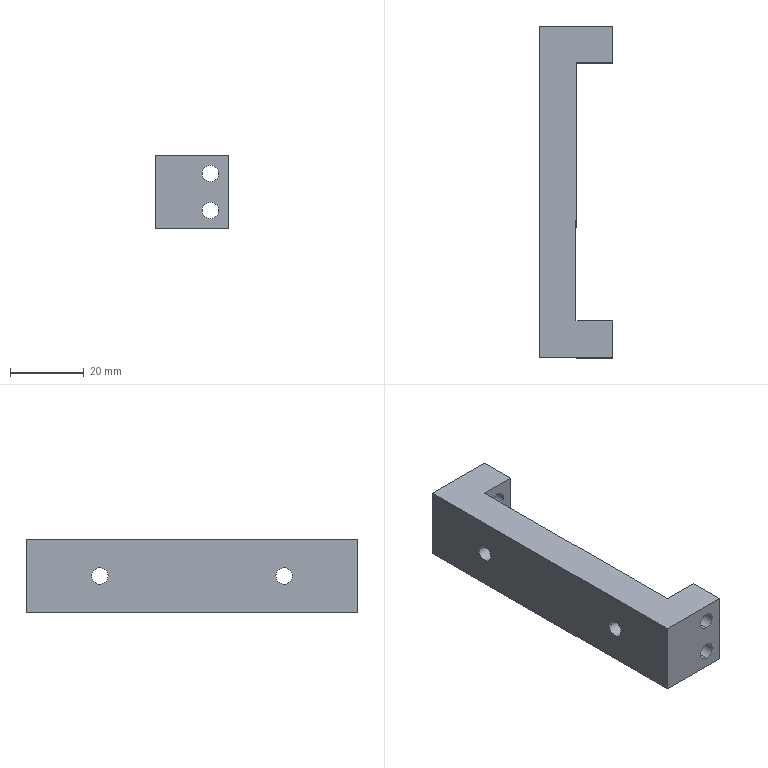Component | SolidWorks | U-shapedEpoxyBoard-2 | 1 solid | 28 faces | box 20 x 90 x 20 mm | volume 20743 mm3 | cylinder 16 | plane 12 | commonest cylinder face diameters 4.5 x12 8 x4
build123d program:
from build123d import *

# Parameters (mm, degrees)
SKETCH1_W                                       = 20
SKETCH1_H                                       = 20
BOSS_EXTRUDE1_DEPTH                             = 45
SKETCH2_W                                       = 70
SKETCH2_H                                       = 10
CUT_EXTRUDE1_DEPTH                              = 90
M4_HEX_SOCKET_HEAD_CAP_SCREW_CBORE1_D           = 4.5
M4_HEX_SOCKET_HEAD_CAP_SCREW_CBORE1_DEPTH       = 12.1
M4_HEX_SOCKET_HEAD_CAP_SCREW_CBORE1_CBORE_D     = 8
M4_HEX_SOCKET_HEAD_CAP_SCREW_CBORE1_CBORE_DEPTH = 4.4
M4_HEX_SOCKET_HEAD_CAP_SCREW_CBORE1_TIP         = 1.352
SKETCH4_R                                       = 2.25
CUT_EXTRUDE2_DEPTH                              = 90


with BuildPart() as part:
    # Sketch1 → Boss-Extrude1 (new, symmetric)
    with BuildSketch(Plane.XY):
        Rectangle(SKETCH1_W, SKETCH1_H)
    extrude(amount=BOSS_EXTRUDE1_DEPTH, both=True)

    # Sketch2 → Cut-Extrude1 (cut)
    with BuildSketch(Plane(origin=(10, 0, 0), x_dir=(0, 0, -1), z_dir=(1, 0, 0))):
        with Locations((0, -5)):
            Rectangle(SKETCH2_W, SKETCH2_H)
    extrude(amount=-CUT_EXTRUDE1_DEPTH, mode=Mode.SUBTRACT)

    # M4 Hex Socket Head Cap Screw CBORE1
    with Locations(Plane(origin=(0, 0, 25), x_dir=(0, 0, -1), z_dir=(0, -1, 0))):
        with Locations((0, 0), (50, 0)):
            CounterBoreHole(M4_HEX_SOCKET_HEAD_CAP_SCREW_CBORE1_D / 2, M4_HEX_SOCKET_HEAD_CAP_SCREW_CBORE1_CBORE_D / 2, M4_HEX_SOCKET_HEAD_CAP_SCREW_CBORE1_CBORE_DEPTH, depth=M4_HEX_SOCKET_HEAD_CAP_SCREW_CBORE1_DEPTH)
            with Locations((0, 0, -(M4_HEX_SOCKET_HEAD_CAP_SCREW_CBORE1_DEPTH + M4_HEX_SOCKET_HEAD_CAP_SCREW_CBORE1_TIP / 2))):  # 118° drill point
                Cone(0, M4_HEX_SOCKET_HEAD_CAP_SCREW_CBORE1_D / 2, M4_HEX_SOCKET_HEAD_CAP_SCREW_CBORE1_TIP, mode=Mode.SUBTRACT)

    # Sketch4 → Cut-Extrude2 (cut)
    with BuildSketch(Plane(origin=(0, 0, -45), x_dir=(-1, 0, 0), z_dir=(0, 0, -1))):
        with Locations((-5, -5)):
            Circle(SKETCH4_R)
        with Locations((5, -5)):
            Circle(SKETCH4_R)
    extrude(amount=-CUT_EXTRUDE2_DEPTH, mode=Mode.SUBTRACT)


solid = part.part

# Placed as in the assembly
solid = solid.moved(Location((-33.341, 37.185, -41.775), (90, 0, 90)))
STEP:
#1=COLOUR_RGB('',0.7922,0.8196,0.9333);
#2=FILL_AREA_STYLE_COLOUR('',#1);
#3=FILL_AREA_STYLE('',(#2));
#4=SURFACE_STYLE_FILL_AREA(#3);
#5=SURFACE_SIDE_STYLE('',(#4));
#6=SURFACE_STYLE_USAGE(.BOTH.,#5);
#7=PRESENTATION_STYLE_ASSIGNMENT((#6));
#8=CARTESIAN_POINT('',(-1.116,-0.3077,-1.753));
#9=VERTEX_POINT('',#8);
#10=CARTESIAN_POINT('',(-1.116,-0.3077,-1.93));
#11=VERTEX_POINT('',#10);
#12=CARTESIAN_POINT('',(-1.116,-0.3077,-1.842));
#13=DIRECTION('',(0.,1.,-0.));
#14=DIRECTION('',(0.,0.,-1.));
#15=AXIS2_PLACEMENT_3D('',#12,#13,#14);
#16=CIRCLE('',#15,0.08858);
#17=EDGE_CURVE('',#9,#11,#16,.T.);
#18=ORIENTED_EDGE('',*,*,#17,.F.);
#19=CARTESIAN_POINT('',(-1.116,0.08603,-1.753));
#20=VERTEX_POINT('',#19);
#21=CARTESIAN_POINT('',(-1.116,-0.3077,-1.753));
#22=DIRECTION('',(0.,1.,-0.));
#23=VECTOR('',#22,39.37);
#24=LINE('',#21,#23);
#25=EDGE_CURVE('',#9,#20,#24,.T.);
#26=ORIENTED_EDGE('',*,*,#25,.T.);
#27=CARTESIAN_POINT('',(-1.116,0.08603,-1.93));
#28=VERTEX_POINT('',#27);
#29=CARTESIAN_POINT('',(-1.116,0.08603,-1.842));
#30=DIRECTION('',(-0.,-1.,0.));
#31=DIRECTION('',(0.,0.,1.));
#32=AXIS2_PLACEMENT_3D('',#29,#30,#31);
#33=CIRCLE('',#32,0.08858);
#34=EDGE_CURVE('',#28,#20,#33,.T.);
#35=ORIENTED_EDGE('',*,*,#34,.F.);
#36=CARTESIAN_POINT('',(-1.116,-0.3077,-1.93));
#37=DIRECTION('',(0.,1.,-0.));
#38=VECTOR('',#37,39.37);
#39=LINE('',#36,#38);
#40=EDGE_CURVE('',#11,#28,#39,.T.);
#41=ORIENTED_EDGE('',*,*,#40,.F.);
#42=EDGE_LOOP('',(#18,#26,#35,#41));
#43=FACE_OUTER_BOUND('',#42,.T.);
#44=CARTESIAN_POINT('',(-1.116,-0.3077,-1.842));
#45=DIRECTION('',(0.,1.,-0.));
#46=DIRECTION('',(0.,0.,-1.));
#47=AXIS2_PLACEMENT_3D('',#44,#45,#46);
#48=CYLINDRICAL_SURFACE('',#47,0.08858);
#49=ADVANCED_FACE('',(#43),#48,.F.);
#50=CARTESIAN_POINT('',(-1.116,2.842,-1.753));
#51=VERTEX_POINT('',#50);
#52=CARTESIAN_POINT('',(-1.116,2.842,-1.93));
#53=VERTEX_POINT('',#52);
#54=CARTESIAN_POINT('',(-1.116,2.842,-1.842));
#55=DIRECTION('',(0.,1.,-0.));
#56=DIRECTION('',(0.,0.,-1.));
#57=AXIS2_PLACEMENT_3D('',#54,#55,#56);
#58=CIRCLE('',#57,0.08858);
#59=EDGE_CURVE('',#51,#53,#58,.T.);
#60=ORIENTED_EDGE('',*,*,#59,.F.);
#61=CARTESIAN_POINT('',(-1.116,3.236,-1.753));
#62=VERTEX_POINT('',#61);
#63=CARTESIAN_POINT('',(-1.116,-0.3077,-1.753));
#64=DIRECTION('',(0.,1.,-0.));
#65=VECTOR('',#64,39.37);
#66=LINE('',#63,#65);
#67=EDGE_CURVE('',#51,#62,#66,.T.);
#68=ORIENTED_EDGE('',*,*,#67,.T.);
#69=CARTESIAN_POINT('',(-1.116,3.236,-1.93));
#70=VERTEX_POINT('',#69);
#71=CARTESIAN_POINT('',(-1.116,3.236,-1.842));
#72=DIRECTION('',(0.,1.,-0.));
#73=DIRECTION('',(0.,0.,-1.));
#74=AXIS2_PLACEMENT_3D('',#71,#72,#73);
#75=CIRCLE('',#74,0.08858);
#76=EDGE_CURVE('',#62,#70,#75,.T.);
#77=ORIENTED_EDGE('',*,*,#76,.T.);
#78=CARTESIAN_POINT('',(-1.116,-0.3077,-1.93));
#79=DIRECTION('',(0.,1.,-0.));
#80=VECTOR('',#79,39.37);
#81=LINE('',#78,#80);
#82=EDGE_CURVE('',#53,#70,#81,.T.);
#83=ORIENTED_EDGE('',*,*,#82,.F.);
#84=EDGE_LOOP('',(#60,#68,#77,#83));
#85=FACE_OUTER_BOUND('',#84,.T.);
#86=CARTESIAN_POINT('',(-1.116,-0.3077,-1.842));
#87=DIRECTION('',(0.,1.,-0.));
#88=DIRECTION('',(0.,0.,-1.));
#89=AXIS2_PLACEMENT_3D('',#86,#87,#88);
#90=CYLINDRICAL_SURFACE('',#89,0.08858);
#91=ADVANCED_FACE('',(#85),#90,.F.);
#92=CARTESIAN_POINT('',(-1.116,-0.3077,-1.359));
#93=VERTEX_POINT('',#92);
#94=CARTESIAN_POINT('',(-1.116,-0.3077,-1.536));
#95=VERTEX_POINT('',#94);
#96=CARTESIAN_POINT('',(-1.116,-0.3077,-1.448));
#97=DIRECTION('',(0.,1.,-0.));
#98=DIRECTION('',(0.,0.,-1.));
#99=AXIS2_PLACEMENT_3D('',#96,#97,#98);
#100=CIRCLE('',#99,0.08858);
#101=EDGE_CURVE('',#93,#95,#100,.T.);
#102=ORIENTED_EDGE('',*,*,#101,.F.);
#103=CARTESIAN_POINT('',(-1.116,0.08603,-1.359));
#104=VERTEX_POINT('',#103);
#105=CARTESIAN_POINT('',(-1.116,-0.3077,-1.359));
#106=DIRECTION('',(0.,1.,-0.));
#107=VECTOR('',#106,39.37);
#108=LINE('',#105,#107);
#109=EDGE_CURVE('',#93,#104,#108,.T.);
#110=ORIENTED_EDGE('',*,*,#109,.T.);
#111=CARTESIAN_POINT('',(-1.116,0.08603,-1.536));
#112=VERTEX_POINT('',#111);
#113=CARTESIAN_POINT('',(-1.116,0.08603,-1.448));
#114=DIRECTION('',(-0.,-1.,0.));
#115=DIRECTION('',(0.,0.,1.));
#116=AXIS2_PLACEMENT_3D('',#113,#114,#115);
#117=CIRCLE('',#116,0.08858);
#118=EDGE_CURVE('',#112,#104,#117,.T.);
#119=ORIENTED_EDGE('',*,*,#118,.F.);
#120=CARTESIAN_POINT('',(-1.116,-0.3077,-1.536));
#121=DIRECTION('',(0.,1.,-0.));
#122=VECTOR('',#121,39.37);
#123=LINE('',#120,#122);
#124=EDGE_CURVE('',#95,#112,#123,.T.);
#125=ORIENTED_EDGE('',*,*,#124,.F.);
#126=EDGE_LOOP('',(#102,#110,#119,#125));
#127=FACE_OUTER_BOUND('',#126,.T.);
#128=CARTESIAN_POINT('',(-1.116,-0.3077,-1.448));
#129=DIRECTION('',(0.,1.,-0.));
#130=DIRECTION('',(0.,0.,-1.));
#131=AXIS2_PLACEMENT_3D('',#128,#129,#130);
#132=CYLINDRICAL_SURFACE('',#131,0.08858);
#133=ADVANCED_FACE('',(#127),#132,.F.);
#134=CARTESIAN_POINT('',(-1.116,2.842,-1.359));
#135=VERTEX_POINT('',#134);
#136=CARTESIAN_POINT('',(-1.116,2.842,-1.536));
#137=VERTEX_POINT('',#136);
#138=CARTESIAN_POINT('',(-1.116,2.842,-1.448));
#139=DIRECTION('',(0.,1.,-0.));
#140=DIRECTION('',(0.,0.,-1.));
#141=AXIS2_PLACEMENT_3D('',#138,#139,#140);
#142=CIRCLE('',#141,0.08858);
#143=EDGE_CURVE('',#135,#137,#142,.T.);
#144=ORIENTED_EDGE('',*,*,#143,.F.);
#145=CARTESIAN_POINT('',(-1.116,3.236,-1.359));
#146=VERTEX_POINT('',#145);
#147=CARTESIAN_POINT('',(-1.116,-0.3077,-1.359));
#148=DIRECTION('',(0.,1.,-0.));
#149=VECTOR('',#148,39.37);
#150=LINE('',#147,#149);
#151=EDGE_CURVE('',#135,#146,#150,.T.);
#152=ORIENTED_EDGE('',*,*,#151,.T.);
#153=CARTESIAN_POINT('',(-1.116,3.236,-1.536));
#154=VERTEX_POINT('',#153);
#155=CARTESIAN_POINT('',(-1.116,3.236,-1.448));
#156=DIRECTION('',(0.,1.,-0.));
#157=DIRECTION('',(0.,0.,-1.));
#158=AXIS2_PLACEMENT_3D('',#155,#156,#157);
#159=CIRCLE('',#158,0.08858);
#160=EDGE_CURVE('',#146,#154,#159,.T.);
#161=ORIENTED_EDGE('',*,*,#160,.T.);
#162=CARTESIAN_POINT('',(-1.116,-0.3077,-1.536));
#163=DIRECTION('',(0.,1.,-0.));
#164=VECTOR('',#163,39.37);
#165=LINE('',#162,#164);
#166=EDGE_CURVE('',#137,#154,#165,.T.);
#167=ORIENTED_EDGE('',*,*,#166,.F.);
#168=EDGE_LOOP('',(#144,#152,#161,#167));
#169=FACE_OUTER_BOUND('',#168,.T.);
#170=CARTESIAN_POINT('',(-1.116,-0.3077,-1.448));
#171=DIRECTION('',(0.,1.,-0.));
#172=DIRECTION('',(0.,0.,-1.));
#173=AXIS2_PLACEMENT_3D('',#170,#171,#172);
#174=CYLINDRICAL_SURFACE('',#173,0.08858);
#175=ADVANCED_FACE('',(#169),#174,.F.);
#176=CARTESIAN_POINT('',(-1.486,0.3223,-1.645));
#177=VERTEX_POINT('',#176);
#178=CARTESIAN_POINT('',(-1.486,0.6372,-1.645));
#179=VERTEX_POINT('',#178);
#180=CARTESIAN_POINT('',(-1.486,0.4797,-1.645));
#181=DIRECTION('',(1.,-0.,-0.));
#182=DIRECTION('',(0.,1.,0.));
#183=AXIS2_PLACEMENT_3D('',#180,#181,#182);
#184=CIRCLE('',#183,0.1575);
#185=EDGE_CURVE('',#177,#179,#184,.T.);
#186=ORIENTED_EDGE('',*,*,#185,.F.);
#187=CARTESIAN_POINT('',(-1.313,0.3223,-1.645));
#188=VERTEX_POINT('',#187);
#189=CARTESIAN_POINT('',(-1.313,0.3223,-1.645));
#190=DIRECTION('',(1.,-0.,-0.));
#191=VECTOR('',#190,39.37);
#192=LINE('',#189,#191);
#193=EDGE_CURVE('',#177,#188,#192,.T.);
#194=ORIENTED_EDGE('',*,*,#193,.T.);
#195=CARTESIAN_POINT('',(-1.313,0.6372,-1.645));
#196=VERTEX_POINT('',#195);
#197=CARTESIAN_POINT('',(-1.313,0.4797,-1.645));
#198=DIRECTION('',(1.,-0.,-0.));
#199=DIRECTION('',(0.,1.,0.));
#200=AXIS2_PLACEMENT_3D('',#197,#198,#199);
#201=CIRCLE('',#200,0.1575);
#202=EDGE_CURVE('',#188,#196,#201,.T.);
#203=ORIENTED_EDGE('',*,*,#202,.T.);
#204=CARTESIAN_POINT('',(-1.313,0.6372,-1.645));
#205=DIRECTION('',(1.,-0.,-0.));
#206=VECTOR('',#205,39.37);
#207=LINE('',#204,#206);
#208=EDGE_CURVE('',#179,#196,#207,.T.);
#209=ORIENTED_EDGE('',*,*,#208,.F.);
#210=EDGE_LOOP('',(#186,#194,#203,#209));
#211=FACE_OUTER_BOUND('',#210,.T.);
#212=CARTESIAN_POINT('',(-1.313,0.4797,-1.645));
#213=DIRECTION('',(1.,-0.,-0.));
#214=DIRECTION('',(0.,1.,0.));
#215=AXIS2_PLACEMENT_3D('',#212,#213,#214);
#216=CYLINDRICAL_SURFACE('',#215,0.1575);
#217=ADVANCED_FACE('',(#211),#216,.F.);
#218=CARTESIAN_POINT('',(-1.706,0.3912,-1.645));
#219=VERTEX_POINT('',#218);
#220=CARTESIAN_POINT('',(-1.706,0.5683,-1.645));
#221=VERTEX_POINT('',#220);
#222=CARTESIAN_POINT('',(-1.706,0.4797,-1.645));
#223=DIRECTION('',(1.,-0.,-0.));
#224=DIRECTION('',(0.,1.,0.));
#225=AXIS2_PLACEMENT_3D('',#222,#223,#224);
#226=CIRCLE('',#225,0.08858);
#227=EDGE_CURVE('',#219,#221,#226,.T.);
#228=ORIENTED_EDGE('',*,*,#227,.F.);
#229=CARTESIAN_POINT('',(-1.486,0.3912,-1.645));
#230=VERTEX_POINT('',#229);
#231=CARTESIAN_POINT('',(-1.313,0.3912,-1.645));
#232=DIRECTION('',(1.,-0.,-0.));
#233=VECTOR('',#232,39.37);
#234=LINE('',#231,#233);
#235=EDGE_CURVE('',#219,#230,#234,.T.);
#236=ORIENTED_EDGE('',*,*,#235,.T.);
#237=CARTESIAN_POINT('',(-1.486,0.5683,-1.645));
#238=VERTEX_POINT('',#237);
#239=CARTESIAN_POINT('',(-1.486,0.4797,-1.645));
#240=DIRECTION('',(1.,-0.,-0.));
#241=DIRECTION('',(0.,1.,0.));
#242=AXIS2_PLACEMENT_3D('',#239,#240,#241);
#243=CIRCLE('',#242,0.08858);
#244=EDGE_CURVE('',#230,#238,#243,.T.);
#245=ORIENTED_EDGE('',*,*,#244,.T.);
#246=CARTESIAN_POINT('',(-1.313,0.5683,-1.645));
#247=DIRECTION('',(1.,-0.,-0.));
#248=VECTOR('',#247,39.37);
#249=LINE('',#246,#248);
#250=EDGE_CURVE('',#221,#238,#249,.T.);
#251=ORIENTED_EDGE('',*,*,#250,.F.);
#252=EDGE_LOOP('',(#228,#236,#245,#251));
#253=FACE_OUTER_BOUND('',#252,.T.);
#254=CARTESIAN_POINT('',(-1.313,0.4797,-1.645));
#255=DIRECTION('',(1.,-0.,-0.));
#256=DIRECTION('',(0.,1.,0.));
#257=AXIS2_PLACEMENT_3D('',#254,#255,#256);
#258=CYLINDRICAL_SURFACE('',#257,0.08858);
#259=ADVANCED_FACE('',(#253),#258,.F.);
#260=CARTESIAN_POINT('',(-1.486,2.291,-1.645));
#261=VERTEX_POINT('',#260);
#262=CARTESIAN_POINT('',(-1.486,2.606,-1.645));
#263=VERTEX_POINT('',#262);
#264=CARTESIAN_POINT('',(-1.486,2.448,-1.645));
#265=DIRECTION('',(1.,-0.,-0.));
#266=DIRECTION('',(0.,1.,0.));
#267=AXIS2_PLACEMENT_3D('',#264,#265,#266);
#268=CIRCLE('',#267,0.1575);
#269=EDGE_CURVE('',#261,#263,#268,.T.);
#270=ORIENTED_EDGE('',*,*,#269,.F.);
#271=CARTESIAN_POINT('',(-1.313,2.291,-1.645));
#272=VERTEX_POINT('',#271);
#273=CARTESIAN_POINT('',(-1.313,2.291,-1.645));
#274=DIRECTION('',(1.,-0.,-0.));
#275=VECTOR('',#274,39.37);
#276=LINE('',#273,#275);
#277=EDGE_CURVE('',#261,#272,#276,.T.);
#278=ORIENTED_EDGE('',*,*,#277,.T.);
#279=CARTESIAN_POINT('',(-1.313,2.606,-1.645));
#280=VERTEX_POINT('',#279);
#281=CARTESIAN_POINT('',(-1.313,2.448,-1.645));
#282=DIRECTION('',(1.,-0.,-0.));
#283=DIRECTION('',(0.,1.,0.));
#284=AXIS2_PLACEMENT_3D('',#281,#282,#283);
#285=CIRCLE('',#284,0.1575);
#286=EDGE_CURVE('',#272,#280,#285,.T.);
#287=ORIENTED_EDGE('',*,*,#286,.T.);
#288=CARTESIAN_POINT('',(-1.313,2.606,-1.645));
#289=DIRECTION('',(1.,-0.,-0.));
#290=VECTOR('',#289,39.37);
#291=LINE('',#288,#290);
#292=EDGE_CURVE('',#263,#280,#291,.T.);
#293=ORIENTED_EDGE('',*,*,#292,.F.);
#294=EDGE_LOOP('',(#270,#278,#287,#293));
#295=FACE_OUTER_BOUND('',#294,.T.);
#296=CARTESIAN_POINT('',(-1.313,2.448,-1.645));
#297=DIRECTION('',(1.,-0.,-0.));
#298=DIRECTION('',(0.,1.,0.));
#299=AXIS2_PLACEMENT_3D('',#296,#297,#298);
#300=CYLINDRICAL_SURFACE('',#299,0.1575);
#301=ADVANCED_FACE('',(#295),#300,.F.);
#302=CARTESIAN_POINT('',(-1.706,2.36,-1.645));
#303=VERTEX_POINT('',#302);
#304=CARTESIAN_POINT('',(-1.706,2.537,-1.645));
#305=VERTEX_POINT('',#304);
#306=CARTESIAN_POINT('',(-1.706,2.448,-1.645));
#307=DIRECTION('',(1.,-0.,-0.));
#308=DIRECTION('',(0.,1.,0.));
#309=AXIS2_PLACEMENT_3D('',#306,#307,#308);
#310=CIRCLE('',#309,0.08858);
#311=EDGE_CURVE('',#303,#305,#310,.T.);
#312=ORIENTED_EDGE('',*,*,#311,.F.);
#313=CARTESIAN_POINT('',(-1.486,2.36,-1.645));
#314=VERTEX_POINT('',#313);
#315=CARTESIAN_POINT('',(-1.313,2.36,-1.645));
#316=DIRECTION('',(1.,-0.,-0.));
#317=VECTOR('',#316,39.37);
#318=LINE('',#315,#317);
#319=EDGE_CURVE('',#303,#314,#318,.T.);
#320=ORIENTED_EDGE('',*,*,#319,.T.);
#321=CARTESIAN_POINT('',(-1.486,2.537,-1.645));
#322=VERTEX_POINT('',#321);
#323=CARTESIAN_POINT('',(-1.486,2.448,-1.645));
#324=DIRECTION('',(1.,-0.,-0.));
#325=DIRECTION('',(0.,1.,0.));
#326=AXIS2_PLACEMENT_3D('',#323,#324,#325);
#327=CIRCLE('',#326,0.08858);
#328=EDGE_CURVE('',#314,#322,#327,.T.);
#329=ORIENTED_EDGE('',*,*,#328,.T.);
#330=CARTESIAN_POINT('',(-1.313,2.537,-1.645));
#331=DIRECTION('',(1.,-0.,-0.));
#332=VECTOR('',#331,39.37);
#333=LINE('',#330,#332);
#334=EDGE_CURVE('',#305,#322,#333,.T.);
#335=ORIENTED_EDGE('',*,*,#334,.F.);
#336=EDGE_LOOP('',(#312,#320,#329,#335));
#337=FACE_OUTER_BOUND('',#336,.T.);
#338=CARTESIAN_POINT('',(-1.313,2.448,-1.645));
#339=DIRECTION('',(1.,-0.,-0.));
#340=DIRECTION('',(0.,1.,0.));
#341=AXIS2_PLACEMENT_3D('',#338,#339,#340);
#342=CYLINDRICAL_SURFACE('',#341,0.08858);
#343=ADVANCED_FACE('',(#337),#342,.F.);
#344=CARTESIAN_POINT('',(-0.919,-0.3077,-2.038));
#345=VERTEX_POINT('',#344);
#346=CARTESIAN_POINT('',(-0.919,0.08603,-2.038));
#347=VERTEX_POINT('',#346);
#348=CARTESIAN_POINT('',(-0.919,-0.3077,-2.038));
#349=DIRECTION('',(0.,1.,-0.));
#350=VECTOR('',#349,39.37);
#351=LINE('',#348,#350);
#352=EDGE_CURVE('',#345,#347,#351,.T.);
#353=ORIENTED_EDGE('',*,*,#352,.T.);
#354=CARTESIAN_POINT('',(-0.919,0.08603,-1.251));
#355=VERTEX_POINT('',#354);
#356=CARTESIAN_POINT('',(-0.919,0.08603,-4.794));
#357=DIRECTION('',(0.,0.,1.));
#358=VECTOR('',#357,39.37);
#359=LINE('',#356,#358);
#360=EDGE_CURVE('',#347,#355,#359,.T.);
#361=ORIENTED_EDGE('',*,*,#360,.T.);
#362=CARTESIAN_POINT('',(-0.919,-0.3077,-1.251));
#363=VERTEX_POINT('',#362);
#364=CARTESIAN_POINT('',(-0.919,-0.3077,-1.251));
#365=DIRECTION('',(0.,1.,-0.));
#366=VECTOR('',#365,39.37);
#367=LINE('',#364,#366);
#368=EDGE_CURVE('',#363,#355,#367,.T.);
#369=ORIENTED_EDGE('',*,*,#368,.F.);
#370=CARTESIAN_POINT('',(-0.919,-0.3077,-2.038));
#371=DIRECTION('',(0.,0.,1.));
#372=VECTOR('',#371,39.37);
#373=LINE('',#370,#372);
#374=EDGE_CURVE('',#345,#363,#373,.T.);
#375=ORIENTED_EDGE('',*,*,#374,.F.);
#376=EDGE_LOOP('',(#353,#361,#369,#375));
#377=FACE_OUTER_BOUND('',#376,.T.);
#378=CARTESIAN_POINT('',(-0.919,-0.3077,-2.038));
#379=DIRECTION('',(-1.,0.,0.));
#380=DIRECTION('',(-0.,-1.,0.));
#381=AXIS2_PLACEMENT_3D('',#378,#379,#380);
#382=PLANE('',#381);
#383=ADVANCED_FACE('',(#377),#382,.F.);
#384=CARTESIAN_POINT('',(-1.313,2.842,-2.038));
#385=VERTEX_POINT('',#384);
#386=CARTESIAN_POINT('',(-1.313,0.08603,-2.038));
#387=VERTEX_POINT('',#386);
#388=CARTESIAN_POINT('',(-1.313,-0.3077,-2.038));
#389=DIRECTION('',(-0.,-1.,0.));
#390=VECTOR('',#389,39.37);
#391=LINE('',#388,#390);
#392=EDGE_CURVE('',#385,#387,#391,.T.);
#393=ORIENTED_EDGE('',*,*,#392,.T.);
#394=CARTESIAN_POINT('',(-1.706,0.08603,-2.038));
#395=DIRECTION('',(1.,-0.,-0.));
#396=VECTOR('',#395,39.37);
#397=LINE('',#394,#396);
#398=EDGE_CURVE('',#387,#347,#397,.T.);
#399=ORIENTED_EDGE('',*,*,#398,.T.);
#400=ORIENTED_EDGE('',*,*,#352,.F.);
#401=CARTESIAN_POINT('',(-1.706,-0.3077,-2.038));
#402=VERTEX_POINT('',#401);
#403=CARTESIAN_POINT('',(-1.706,-0.3077,-2.038));
#404=DIRECTION('',(1.,-0.,-0.));
#405=VECTOR('',#404,39.37);
#406=LINE('',#403,#405);
#407=EDGE_CURVE('',#402,#345,#406,.T.);
#408=ORIENTED_EDGE('',*,*,#407,.F.);
#409=CARTESIAN_POINT('',(-1.706,3.236,-2.038));
#410=VERTEX_POINT('',#409);
#411=CARTESIAN_POINT('',(-1.706,-0.3077,-2.038));
#412=DIRECTION('',(0.,1.,-0.));
#413=VECTOR('',#412,39.37);
#414=LINE('',#411,#413);
#415=EDGE_CURVE('',#402,#410,#414,.T.);
#416=ORIENTED_EDGE('',*,*,#415,.T.);
#417=CARTESIAN_POINT('',(-0.919,3.236,-2.038));
#418=VERTEX_POINT('',#417);
#419=CARTESIAN_POINT('',(-1.706,3.236,-2.038));
#420=DIRECTION('',(1.,-0.,-0.));
#421=VECTOR('',#420,39.37);
#422=LINE('',#419,#421);
#423=EDGE_CURVE('',#410,#418,#422,.T.);
#424=ORIENTED_EDGE('',*,*,#423,.T.);
#425=CARTESIAN_POINT('',(-0.919,2.842,-2.038));
#426=VERTEX_POINT('',#425);
#427=CARTESIAN_POINT('',(-0.919,-0.3077,-2.038));
#428=DIRECTION('',(0.,1.,-0.));
#429=VECTOR('',#428,39.37);
#430=LINE('',#427,#429);
#431=EDGE_CURVE('',#426,#418,#430,.T.);
#432=ORIENTED_EDGE('',*,*,#431,.F.);
#433=CARTESIAN_POINT('',(-1.706,2.842,-2.038));
#434=DIRECTION('',(-1.,0.,0.));
#435=VECTOR('',#434,39.37);
#436=LINE('',#433,#435);
#437=EDGE_CURVE('',#426,#385,#436,.T.);
#438=ORIENTED_EDGE('',*,*,#437,.T.);
#439=EDGE_LOOP('',(#393,#399,#400,#408,#416,#424,#432,#438));
#440=FACE_OUTER_BOUND('',#439,.T.);
#441=CARTESIAN_POINT('',(-1.706,-0.3077,-2.038));
#442=DIRECTION('',(0.,0.,1.));
#443=DIRECTION('',(-1.,0.,0.));
#444=AXIS2_PLACEMENT_3D('',#441,#442,#443);
#445=PLANE('',#444);
#446=ADVANCED_FACE('',(#440),#445,.F.);
#447=CARTESIAN_POINT('',(-0.919,2.842,-1.251));
#448=VERTEX_POINT('',#447);
#449=CARTESIAN_POINT('',(-0.919,3.236,-1.251));
#450=VERTEX_POINT('',#449);
#451=CARTESIAN_POINT('',(-0.919,-0.3077,-1.251));
#452=DIRECTION('',(0.,1.,-0.));
#453=VECTOR('',#452,39.37);
#454=LINE('',#451,#453);
#455=EDGE_CURVE('',#448,#450,#454,.T.);
#456=ORIENTED_EDGE('',*,*,#455,.F.);
#457=CARTESIAN_POINT('',(-0.919,2.842,-4.794));
#458=DIRECTION('',(0.,0.,1.));
#459=VECTOR('',#458,39.37);
#460=LINE('',#457,#459);
#461=EDGE_CURVE('',#426,#448,#460,.T.);
#462=ORIENTED_EDGE('',*,*,#461,.F.);
#463=ORIENTED_EDGE('',*,*,#431,.T.);
#464=CARTESIAN_POINT('',(-0.919,3.236,-2.038));
#465=DIRECTION('',(0.,0.,1.));
#466=VECTOR('',#465,39.37);
#467=LINE('',#464,#466);
#468=EDGE_CURVE('',#418,#450,#467,.T.);
#469=ORIENTED_EDGE('',*,*,#468,.T.);
#470=EDGE_LOOP('',(#456,#462,#463,#469));
#471=FACE_OUTER_BOUND('',#470,.T.);
#472=CARTESIAN_POINT('',(-0.919,-0.3077,-2.038));
#473=DIRECTION('',(-1.,0.,0.));
#474=DIRECTION('',(-0.,-1.,0.));
#475=AXIS2_PLACEMENT_3D('',#472,#473,#474);
#476=PLANE('',#475);
#477=ADVANCED_FACE('',(#471),#476,.F.);
#478=ORIENTED_EDGE('',*,*,#368,.T.);
#479=CARTESIAN_POINT('',(-1.313,0.08603,-1.251));
#480=VERTEX_POINT('',#479);
#481=CARTESIAN_POINT('',(-0.919,0.08603,-1.251));
#482=DIRECTION('',(1.,-0.,-0.));
#483=VECTOR('',#482,39.37);
#484=LINE('',#481,#483);
#485=EDGE_CURVE('',#480,#355,#484,.T.);
#486=ORIENTED_EDGE('',*,*,#485,.F.);
#487=CARTESIAN_POINT('',(-1.313,2.842,-1.251));
#488=VERTEX_POINT('',#487);
#489=CARTESIAN_POINT('',(-1.313,0.08603,-1.251));
#490=DIRECTION('',(-0.,-1.,0.));
#491=VECTOR('',#490,39.37);
#492=LINE('',#489,#491);
#493=EDGE_CURVE('',#488,#480,#492,.T.);
#494=ORIENTED_EDGE('',*,*,#493,.F.);
#495=CARTESIAN_POINT('',(-0.919,2.842,-1.251));
#496=DIRECTION('',(-1.,0.,0.));
#497=VECTOR('',#496,39.37);
#498=LINE('',#495,#497);
#499=EDGE_CURVE('',#448,#488,#498,.T.);
#500=ORIENTED_EDGE('',*,*,#499,.F.);
#501=ORIENTED_EDGE('',*,*,#455,.T.);
#502=CARTESIAN_POINT('',(-1.706,3.236,-1.251));
#503=VERTEX_POINT('',#502);
#504=CARTESIAN_POINT('',(-1.706,3.236,-1.251));
#505=DIRECTION('',(-1.,0.,0.));
#506=VECTOR('',#505,39.37);
#507=LINE('',#504,#506);
#508=EDGE_CURVE('',#450,#503,#507,.T.);
#509=ORIENTED_EDGE('',*,*,#508,.T.);
#510=CARTESIAN_POINT('',(-1.706,-0.3077,-1.251));
#511=VERTEX_POINT('',#510);
#512=CARTESIAN_POINT('',(-1.706,-0.3077,-1.251));
#513=DIRECTION('',(0.,1.,-0.));
#514=VECTOR('',#513,39.37);
#515=LINE('',#512,#514);
#516=EDGE_CURVE('',#511,#503,#515,.T.);
#517=ORIENTED_EDGE('',*,*,#516,.F.);
#518=CARTESIAN_POINT('',(-1.706,-0.3077,-1.251));
#519=DIRECTION('',(-1.,0.,0.));
#520=VECTOR('',#519,39.37);
#521=LINE('',#518,#520);
#522=EDGE_CURVE('',#363,#511,#521,.T.);
#523=ORIENTED_EDGE('',*,*,#522,.F.);
#524=EDGE_LOOP('',(#478,#486,#494,#500,#501,#509,#517,#523));
#525=FACE_OUTER_BOUND('',#524,.T.);
#526=CARTESIAN_POINT('',(-1.706,-0.3077,-1.251));
#527=DIRECTION('',(-0.,-0.,-1.));
#528=DIRECTION('',(-0.,-1.,0.));
#529=AXIS2_PLACEMENT_3D('',#526,#527,#528);
#530=PLANE('',#529);
#531=ADVANCED_FACE('',(#525),#530,.F.);
#532=CARTESIAN_POINT('',(-1.706,0.4797,-1.645));
#533=DIRECTION('',(1.,-0.,-0.));
#534=DIRECTION('',(0.,1.,0.));
#535=AXIS2_PLACEMENT_3D('',#532,#533,#534);
#536=CIRCLE('',#535,0.08858);
#537=EDGE_CURVE('',#221,#219,#536,.T.);
#538=ORIENTED_EDGE('',*,*,#537,.T.);
#539=ORIENTED_EDGE('',*,*,#227,.T.);
#540=EDGE_LOOP('',(#538,#539));
#541=FACE_BOUND('',#540,.T.);
#542=CARTESIAN_POINT('',(-1.706,2.448,-1.645));
#543=DIRECTION('',(1.,-0.,-0.));
#544=DIRECTION('',(0.,1.,0.));
#545=AXIS2_PLACEMENT_3D('',#542,#543,#544);
#546=CIRCLE('',#545,0.08858);
#547=EDGE_CURVE('',#305,#303,#546,.T.);
#548=ORIENTED_EDGE('',*,*,#547,.T.);
#549=ORIENTED_EDGE('',*,*,#311,.T.);
#550=EDGE_LOOP('',(#548,#549));
#551=FACE_BOUND('',#550,.T.);
#552=CARTESIAN_POINT('',(-1.706,3.236,-2.038));
#553=DIRECTION('',(-0.,-0.,-1.));
#554=VECTOR('',#553,39.37);
#555=LINE('',#552,#554);
#556=EDGE_CURVE('',#503,#410,#555,.T.);
#557=ORIENTED_EDGE('',*,*,#556,.T.);
#558=ORIENTED_EDGE('',*,*,#415,.F.);
#559=CARTESIAN_POINT('',(-1.706,-0.3077,-2.038));
#560=DIRECTION('',(-0.,-0.,-1.));
#561=VECTOR('',#560,39.37);
#562=LINE('',#559,#561);
#563=EDGE_CURVE('',#511,#402,#562,.T.);
#564=ORIENTED_EDGE('',*,*,#563,.F.);
#565=ORIENTED_EDGE('',*,*,#516,.T.);
#566=EDGE_LOOP('',(#557,#558,#564,#565));
#567=FACE_OUTER_BOUND('',#566,.T.);
#568=CARTESIAN_POINT('',(-1.706,-0.3077,-2.038));
#569=DIRECTION('',(1.,-0.,-0.));
#570=DIRECTION('',(0.,1.,-0.));
#571=AXIS2_PLACEMENT_3D('',#568,#569,#570);
#572=PLANE('',#571);
#573=ADVANCED_FACE('',(#541,#551,#567),#572,.F.);
#574=CARTESIAN_POINT('',(-1.116,-0.3077,-1.842));
#575=DIRECTION('',(0.,1.,-0.));
#576=DIRECTION('',(0.,0.,-1.));
#577=AXIS2_PLACEMENT_3D('',#574,#575,#576);
#578=CIRCLE('',#577,0.08858);
#579=EDGE_CURVE('',#11,#9,#578,.T.);
#580=ORIENTED_EDGE('',*,*,#579,.T.);
#581=ORIENTED_EDGE('',*,*,#17,.T.);
#582=EDGE_LOOP('',(#580,#581));
#583=FACE_BOUND('',#582,.T.);
#584=CARTESIAN_POINT('',(-1.116,-0.3077,-1.448));
#585=DIRECTION('',(0.,1.,-0.));
#586=DIRECTION('',(0.,0.,-1.));
#587=AXIS2_PLACEMENT_3D('',#584,#585,#586);
#588=CIRCLE('',#587,0.08858);
#589=EDGE_CURVE('',#95,#93,#588,.T.);
#590=ORIENTED_EDGE('',*,*,#589,.T.);
#591=ORIENTED_EDGE('',*,*,#101,.T.);
#592=EDGE_LOOP('',(#590,#591));
#593=FACE_BOUND('',#592,.T.);
#594=ORIENTED_EDGE('',*,*,#407,.T.);
#595=ORIENTED_EDGE('',*,*,#374,.T.);
#596=ORIENTED_EDGE('',*,*,#522,.T.);
#597=ORIENTED_EDGE('',*,*,#563,.T.);
#598=EDGE_LOOP('',(#594,#595,#596,#597));
#599=FACE_OUTER_BOUND('',#598,.T.);
#600=CARTESIAN_POINT('',(-1.313,-0.3077,-1.645));
#601=DIRECTION('',(-0.,-1.,0.));
#602=DIRECTION('',(0.,0.,1.));
#603=AXIS2_PLACEMENT_3D('',#600,#601,#602);
#604=PLANE('',#603);
#605=ADVANCED_FACE('',(#583,#593,#599),#604,.T.);
#606=CARTESIAN_POINT('',(-1.116,3.236,-1.842));
#607=DIRECTION('',(0.,1.,-0.));
#608=DIRECTION('',(0.,0.,-1.));
#609=AXIS2_PLACEMENT_3D('',#606,#607,#608);
#610=CIRCLE('',#609,0.08858);
#611=EDGE_CURVE('',#70,#62,#610,.T.);
#612=ORIENTED_EDGE('',*,*,#611,.F.);
#613=ORIENTED_EDGE('',*,*,#76,.F.);
#614=EDGE_LOOP('',(#612,#613));
#615=FACE_BOUND('',#614,.T.);
#616=CARTESIAN_POINT('',(-1.116,3.236,-1.448));
#617=DIRECTION('',(0.,1.,-0.));
#618=DIRECTION('',(0.,0.,-1.));
#619=AXIS2_PLACEMENT_3D('',#616,#617,#618);
#620=CIRCLE('',#619,0.08858);
#621=EDGE_CURVE('',#154,#146,#620,.T.);
#622=ORIENTED_EDGE('',*,*,#621,.F.);
#623=ORIENTED_EDGE('',*,*,#160,.F.);
#624=EDGE_LOOP('',(#622,#623));
#625=FACE_BOUND('',#624,.T.);
#626=ORIENTED_EDGE('',*,*,#423,.F.);
#627=ORIENTED_EDGE('',*,*,#556,.F.);
#628=ORIENTED_EDGE('',*,*,#508,.F.);
#629=ORIENTED_EDGE('',*,*,#468,.F.);
#630=EDGE_LOOP('',(#626,#627,#628,#629));
#631=FACE_OUTER_BOUND('',#630,.T.);
#632=CARTESIAN_POINT('',(-1.313,3.236,-1.645));
#633=DIRECTION('',(-0.,-1.,0.));
#634=DIRECTION('',(0.,0.,1.));
#635=AXIS2_PLACEMENT_3D('',#632,#633,#634);
#636=PLANE('',#635);
#637=ADVANCED_FACE('',(#615,#625,#631),#636,.F.);
#638=ORIENTED_EDGE('',*,*,#34,.T.);
#639=CARTESIAN_POINT('',(-1.116,0.08603,-1.842));
#640=DIRECTION('',(-0.,-1.,0.));
#641=DIRECTION('',(0.,0.,1.));
#642=AXIS2_PLACEMENT_3D('',#639,#640,#641);
#643=CIRCLE('',#642,0.08858);
#644=EDGE_CURVE('',#20,#28,#643,.T.);
#645=ORIENTED_EDGE('',*,*,#644,.T.);
#646=EDGE_LOOP('',(#638,#645));
#647=FACE_BOUND('',#646,.T.);
#648=ORIENTED_EDGE('',*,*,#118,.T.);
#649=CARTESIAN_POINT('',(-1.116,0.08603,-1.448));
#650=DIRECTION('',(-0.,-1.,0.));
#651=DIRECTION('',(0.,0.,1.));
#652=AXIS2_PLACEMENT_3D('',#649,#650,#651);
#653=CIRCLE('',#652,0.08858);
#654=EDGE_CURVE('',#104,#112,#653,.T.);
#655=ORIENTED_EDGE('',*,*,#654,.T.);
#656=EDGE_LOOP('',(#648,#655));
#657=FACE_BOUND('',#656,.T.);
#658=CARTESIAN_POINT('',(-1.313,0.08603,-4.794));
#659=DIRECTION('',(0.,0.,1.));
#660=VECTOR('',#659,39.37);
#661=LINE('',#658,#660);
#662=EDGE_CURVE('',#387,#480,#661,.T.);
#663=ORIENTED_EDGE('',*,*,#662,.T.);
#664=ORIENTED_EDGE('',*,*,#485,.T.);
#665=ORIENTED_EDGE('',*,*,#360,.F.);
#666=ORIENTED_EDGE('',*,*,#398,.F.);
#667=EDGE_LOOP('',(#663,#664,#665,#666));
#668=FACE_OUTER_BOUND('',#667,.T.);
#669=CARTESIAN_POINT('',(-0.919,0.08603,-4.794));
#670=DIRECTION('',(-0.,-1.,0.));
#671=DIRECTION('',(0.,0.,1.));
#672=AXIS2_PLACEMENT_3D('',#669,#670,#671);
#673=PLANE('',#672);
#674=ADVANCED_FACE('',(#647,#657,#668),#673,.F.);
#675=CARTESIAN_POINT('',(-1.313,0.4797,-1.645));
#676=DIRECTION('',(1.,-0.,-0.));
#677=DIRECTION('',(0.,1.,0.));
#678=AXIS2_PLACEMENT_3D('',#675,#676,#677);
#679=CIRCLE('',#678,0.1575);
#680=EDGE_CURVE('',#196,#188,#679,.T.);
#681=ORIENTED_EDGE('',*,*,#680,.F.);
#682=ORIENTED_EDGE('',*,*,#202,.F.);
#683=EDGE_LOOP('',(#681,#682));
#684=FACE_BOUND('',#683,.T.);
#685=CARTESIAN_POINT('',(-1.313,2.448,-1.645));
#686=DIRECTION('',(1.,-0.,-0.));
#687=DIRECTION('',(0.,1.,0.));
#688=AXIS2_PLACEMENT_3D('',#685,#686,#687);
#689=CIRCLE('',#688,0.1575);
#690=EDGE_CURVE('',#280,#272,#689,.T.);
#691=ORIENTED_EDGE('',*,*,#690,.F.);
#692=ORIENTED_EDGE('',*,*,#286,.F.);
#693=EDGE_LOOP('',(#691,#692));
#694=FACE_BOUND('',#693,.T.);
#695=CARTESIAN_POINT('',(-1.313,2.842,-4.794));
#696=DIRECTION('',(0.,0.,1.));
#697=VECTOR('',#696,39.37);
#698=LINE('',#695,#697);
#699=EDGE_CURVE('',#385,#488,#698,.T.);
#700=ORIENTED_EDGE('',*,*,#699,.T.);
#701=ORIENTED_EDGE('',*,*,#493,.T.);
#702=ORIENTED_EDGE('',*,*,#662,.F.);
#703=ORIENTED_EDGE('',*,*,#392,.F.);
#704=EDGE_LOOP('',(#700,#701,#702,#703));
#705=FACE_OUTER_BOUND('',#704,.T.);
#706=CARTESIAN_POINT('',(-1.313,0.08603,-4.794));
#707=DIRECTION('',(-1.,0.,0.));
#708=DIRECTION('',(-0.,-1.,0.));
#709=AXIS2_PLACEMENT_3D('',#706,#707,#708);
#710=PLANE('',#709);
#711=ADVANCED_FACE('',(#684,#694,#705),#710,.F.);
#712=CARTESIAN_POINT('',(-1.116,2.842,-1.842));
#713=DIRECTION('',(0.,1.,-0.));
#714=DIRECTION('',(0.,0.,-1.));
#715=AXIS2_PLACEMENT_3D('',#712,#713,#714);
#716=CIRCLE('',#715,0.08858);
#717=EDGE_CURVE('',#53,#51,#716,.T.);
#718=ORIENTED_EDGE('',*,*,#717,.T.);
#719=ORIENTED_EDGE('',*,*,#59,.T.);
#720=EDGE_LOOP('',(#718,#719));
#721=FACE_BOUND('',#720,.T.);
#722=CARTESIAN_POINT('',(-1.116,2.842,-1.448));
#723=DIRECTION('',(0.,1.,-0.));
#724=DIRECTION('',(0.,0.,-1.));
#725=AXIS2_PLACEMENT_3D('',#722,#723,#724);
#726=CIRCLE('',#725,0.08858);
#727=EDGE_CURVE('',#137,#135,#726,.T.);
#728=ORIENTED_EDGE('',*,*,#727,.T.);
#729=ORIENTED_EDGE('',*,*,#143,.T.);
#730=EDGE_LOOP('',(#728,#729));
#731=FACE_BOUND('',#730,.T.);
#732=ORIENTED_EDGE('',*,*,#461,.T.);
#733=ORIENTED_EDGE('',*,*,#499,.T.);
#734=ORIENTED_EDGE('',*,*,#699,.F.);
#735=ORIENTED_EDGE('',*,*,#437,.F.);
#736=EDGE_LOOP('',(#732,#733,#734,#735));
#737=FACE_OUTER_BOUND('',#736,.T.);
#738=CARTESIAN_POINT('',(-0.919,2.842,-4.794));
#739=DIRECTION('',(0.,1.,-0.));
#740=DIRECTION('',(-0.,-0.,-1.));
#741=AXIS2_PLACEMENT_3D('',#738,#739,#740);
#742=PLANE('',#741);
#743=ADVANCED_FACE('',(#721,#731,#737),#742,.F.);
#744=ORIENTED_EDGE('',*,*,#319,.F.);
#745=ORIENTED_EDGE('',*,*,#547,.F.);
#746=ORIENTED_EDGE('',*,*,#334,.T.);
#747=CARTESIAN_POINT('',(-1.486,2.448,-1.645));
#748=DIRECTION('',(1.,-0.,-0.));
#749=DIRECTION('',(0.,1.,0.));
#750=AXIS2_PLACEMENT_3D('',#747,#748,#749);
#751=CIRCLE('',#750,0.08858);
#752=EDGE_CURVE('',#322,#314,#751,.T.);
#753=ORIENTED_EDGE('',*,*,#752,.T.);
#754=EDGE_LOOP('',(#744,#745,#746,#753));
#755=FACE_OUTER_BOUND('',#754,.T.);
#756=CARTESIAN_POINT('',(-1.313,2.448,-1.645));
#757=DIRECTION('',(1.,-0.,-0.));
#758=DIRECTION('',(0.,1.,0.));
#759=AXIS2_PLACEMENT_3D('',#756,#757,#758);
#760=CYLINDRICAL_SURFACE('',#759,0.08858);
#761=ADVANCED_FACE('',(#755),#760,.F.);
#762=ORIENTED_EDGE('',*,*,#752,.F.);
#763=ORIENTED_EDGE('',*,*,#328,.F.);
#764=EDGE_LOOP('',(#762,#763));
#765=FACE_BOUND('',#764,.T.);
#766=CARTESIAN_POINT('',(-1.486,2.448,-1.645));
#767=DIRECTION('',(1.,-0.,-0.));
#768=DIRECTION('',(0.,1.,0.));
#769=AXIS2_PLACEMENT_3D('',#766,#767,#768);
#770=CIRCLE('',#769,0.1575);
#771=EDGE_CURVE('',#263,#261,#770,.T.);
#772=ORIENTED_EDGE('',*,*,#771,.T.);
#773=ORIENTED_EDGE('',*,*,#269,.T.);
#774=EDGE_LOOP('',(#772,#773));
#775=FACE_OUTER_BOUND('',#774,.T.);
#776=CARTESIAN_POINT('',(-1.486,2.448,-1.556));
#777=DIRECTION('',(-1.,0.,0.));
#778=DIRECTION('',(-0.,-1.,0.));
#779=AXIS2_PLACEMENT_3D('',#776,#777,#778);
#780=PLANE('',#779);
#781=ADVANCED_FACE('',(#765,#775),#780,.F.);
#782=ORIENTED_EDGE('',*,*,#277,.F.);
#783=ORIENTED_EDGE('',*,*,#771,.F.);
#784=ORIENTED_EDGE('',*,*,#292,.T.);
#785=ORIENTED_EDGE('',*,*,#690,.T.);
#786=EDGE_LOOP('',(#782,#783,#784,#785));
#787=FACE_OUTER_BOUND('',#786,.T.);
#788=CARTESIAN_POINT('',(-1.313,2.448,-1.645));
#789=DIRECTION('',(1.,-0.,-0.));
#790=DIRECTION('',(0.,1.,0.));
#791=AXIS2_PLACEMENT_3D('',#788,#789,#790);
#792=CYLINDRICAL_SURFACE('',#791,0.1575);
#793=ADVANCED_FACE('',(#787),#792,.F.);
#794=ORIENTED_EDGE('',*,*,#235,.F.);
#795=ORIENTED_EDGE('',*,*,#537,.F.);
#796=ORIENTED_EDGE('',*,*,#250,.T.);
#797=CARTESIAN_POINT('',(-1.486,0.4797,-1.645));
#798=DIRECTION('',(1.,-0.,-0.));
#799=DIRECTION('',(0.,1.,0.));
#800=AXIS2_PLACEMENT_3D('',#797,#798,#799);
#801=CIRCLE('',#800,0.08858);
#802=EDGE_CURVE('',#238,#230,#801,.T.);
#803=ORIENTED_EDGE('',*,*,#802,.T.);
#804=EDGE_LOOP('',(#794,#795,#796,#803));
#805=FACE_OUTER_BOUND('',#804,.T.);
#806=CARTESIAN_POINT('',(-1.313,0.4797,-1.645));
#807=DIRECTION('',(1.,-0.,-0.));
#808=DIRECTION('',(0.,1.,0.));
#809=AXIS2_PLACEMENT_3D('',#806,#807,#808);
#810=CYLINDRICAL_SURFACE('',#809,0.08858);
#811=ADVANCED_FACE('',(#805),#810,.F.);
#812=ORIENTED_EDGE('',*,*,#802,.F.);
#813=ORIENTED_EDGE('',*,*,#244,.F.);
#814=EDGE_LOOP('',(#812,#813));
#815=FACE_BOUND('',#814,.T.);
#816=CARTESIAN_POINT('',(-1.486,0.4797,-1.645));
#817=DIRECTION('',(1.,-0.,-0.));
#818=DIRECTION('',(0.,1.,0.));
#819=AXIS2_PLACEMENT_3D('',#816,#817,#818);
#820=CIRCLE('',#819,0.1575);
#821=EDGE_CURVE('',#179,#177,#820,.T.);
#822=ORIENTED_EDGE('',*,*,#821,.T.);
#823=ORIENTED_EDGE('',*,*,#185,.T.);
#824=EDGE_LOOP('',(#822,#823));
#825=FACE_OUTER_BOUND('',#824,.T.);
#826=CARTESIAN_POINT('',(-1.486,0.4797,-1.556));
#827=DIRECTION('',(-1.,0.,0.));
#828=DIRECTION('',(-0.,-1.,0.));
#829=AXIS2_PLACEMENT_3D('',#826,#827,#828);
#830=PLANE('',#829);
#831=ADVANCED_FACE('',(#815,#825),#830,.F.);
#832=ORIENTED_EDGE('',*,*,#193,.F.);
#833=ORIENTED_EDGE('',*,*,#821,.F.);
#834=ORIENTED_EDGE('',*,*,#208,.T.);
#835=ORIENTED_EDGE('',*,*,#680,.T.);
#836=EDGE_LOOP('',(#832,#833,#834,#835));
#837=FACE_OUTER_BOUND('',#836,.T.);
#838=CARTESIAN_POINT('',(-1.313,0.4797,-1.645));
#839=DIRECTION('',(1.,-0.,-0.));
#840=DIRECTION('',(0.,1.,0.));
#841=AXIS2_PLACEMENT_3D('',#838,#839,#840);
#842=CYLINDRICAL_SURFACE('',#841,0.1575);
#843=ADVANCED_FACE('',(#837),#842,.F.);
#844=ORIENTED_EDGE('',*,*,#151,.F.);
#845=ORIENTED_EDGE('',*,*,#727,.F.);
#846=ORIENTED_EDGE('',*,*,#166,.T.);
#847=ORIENTED_EDGE('',*,*,#621,.T.);
#848=EDGE_LOOP('',(#844,#845,#846,#847));
#849=FACE_OUTER_BOUND('',#848,.T.);
#850=CARTESIAN_POINT('',(-1.116,-0.3077,-1.448));
#851=DIRECTION('',(0.,1.,-0.));
#852=DIRECTION('',(0.,0.,-1.));
#853=AXIS2_PLACEMENT_3D('',#850,#851,#852);
#854=CYLINDRICAL_SURFACE('',#853,0.08858);
#855=ADVANCED_FACE('',(#849),#854,.F.);
#856=ORIENTED_EDGE('',*,*,#109,.F.);
#857=ORIENTED_EDGE('',*,*,#589,.F.);
#858=ORIENTED_EDGE('',*,*,#124,.T.);
#859=ORIENTED_EDGE('',*,*,#654,.F.);
#860=EDGE_LOOP('',(#856,#857,#858,#859));
#861=FACE_OUTER_BOUND('',#860,.T.);
#862=CARTESIAN_POINT('',(-1.116,-0.3077,-1.448));
#863=DIRECTION('',(0.,1.,-0.));
#864=DIRECTION('',(0.,0.,-1.));
#865=AXIS2_PLACEMENT_3D('',#862,#863,#864);
#866=CYLINDRICAL_SURFACE('',#865,0.08858);
#867=ADVANCED_FACE('',(#861),#866,.F.);
#868=ORIENTED_EDGE('',*,*,#67,.F.);
#869=ORIENTED_EDGE('',*,*,#717,.F.);
#870=ORIENTED_EDGE('',*,*,#82,.T.);
#871=ORIENTED_EDGE('',*,*,#611,.T.);
#872=EDGE_LOOP('',(#868,#869,#870,#871));
#873=FACE_OUTER_BOUND('',#872,.T.);
#874=CARTESIAN_POINT('',(-1.116,-0.3077,-1.842));
#875=DIRECTION('',(0.,1.,-0.));
#876=DIRECTION('',(0.,0.,-1.));
#877=AXIS2_PLACEMENT_3D('',#874,#875,#876);
#878=CYLINDRICAL_SURFACE('',#877,0.08858);
#879=ADVANCED_FACE('',(#873),#878,.F.);
#880=ORIENTED_EDGE('',*,*,#25,.F.);
#881=ORIENTED_EDGE('',*,*,#579,.F.);
#882=ORIENTED_EDGE('',*,*,#40,.T.);
#883=ORIENTED_EDGE('',*,*,#644,.F.);
#884=EDGE_LOOP('',(#880,#881,#882,#883));
#885=FACE_OUTER_BOUND('',#884,.T.);
#886=CARTESIAN_POINT('',(-1.116,-0.3077,-1.842));
#887=DIRECTION('',(0.,1.,-0.));
#888=DIRECTION('',(0.,0.,-1.));
#889=AXIS2_PLACEMENT_3D('',#886,#887,#888);
#890=CYLINDRICAL_SURFACE('',#889,0.08858);
#891=ADVANCED_FACE('',(#885),#890,.F.);
#892=CLOSED_SHELL('',(#49,#91,#133,#175,#217,#259,#301,#343,#383,#446,#477,#531,#573,#605,#637,#674,#711,#743,#761,#781,#793,#811,#831,#843,#855,#867,#879,#891));
#893=MANIFOLD_SOLID_BREP('',#892);
#894=STYLED_ITEM('',(#7),#893);
#895=PRESENTATION_LAYER_ASSIGNMENT('','',(#894));
#896=(LENGTH_UNIT()NAMED_UNIT(*)SI_UNIT($,.METRE.));
#897=LENGTH_MEASURE_WITH_UNIT(LENGTH_MEASURE(0.0254),#896);
#898=DIMENSIONAL_EXPONENTS(1.,0.,0.,0.,0.,0.,0.);
#899=(CONVERSION_BASED_UNIT('',#897)LENGTH_UNIT()NAMED_UNIT(#898));
#900=UNCERTAINTY_MEASURE_WITH_UNIT(LENGTH_MEASURE(0.00001),#899,'','');
#901=(NAMED_UNIT(*)PLANE_ANGLE_UNIT()SI_UNIT($,.RADIAN.));
#902=(NAMED_UNIT(*)SI_UNIT($,.STERADIAN.)SOLID_ANGLE_UNIT());
#903=(GEOMETRIC_REPRESENTATION_CONTEXT(3)GLOBAL_UNCERTAINTY_ASSIGNED_CONTEXT((#900))GLOBAL_UNIT_ASSIGNED_CONTEXT((#899,#901,#902))REPRESENTATION_CONTEXT('',''));
#904=MECHANICAL_DESIGN_GEOMETRIC_PRESENTATION_REPRESENTATION('',(#894),#903);
#905=CARTESIAN_POINT('',(0.,0.,0.));
#906=DIRECTION('',(0.,0.,1.));
#907=DIRECTION('',(1.,0.,0.));
#908=AXIS2_PLACEMENT_3D('',#905,#906,#907);
#909=(LENGTH_UNIT()NAMED_UNIT(*)SI_UNIT($,.METRE.));
#910=LENGTH_MEASURE_WITH_UNIT(LENGTH_MEASURE(0.0254),#909);
#911=DIMENSIONAL_EXPONENTS(1.,0.,0.,0.,0.,0.,0.);
#912=(CONVERSION_BASED_UNIT('',#910)LENGTH_UNIT()NAMED_UNIT(#911));
#913=UNCERTAINTY_MEASURE_WITH_UNIT(LENGTH_MEASURE(0.00001),#912,'','');
#914=(NAMED_UNIT(*)PLANE_ANGLE_UNIT()SI_UNIT($,.RADIAN.));
#915=(NAMED_UNIT(*)SI_UNIT($,.STERADIAN.)SOLID_ANGLE_UNIT());
#916=(GEOMETRIC_REPRESENTATION_CONTEXT(3)GLOBAL_UNCERTAINTY_ASSIGNED_CONTEXT((#913))GLOBAL_UNIT_ASSIGNED_CONTEXT((#912,#914,#915))REPRESENTATION_CONTEXT('',''));
#917=ADVANCED_BREP_SHAPE_REPRESENTATION('',(#893,#908),#916);